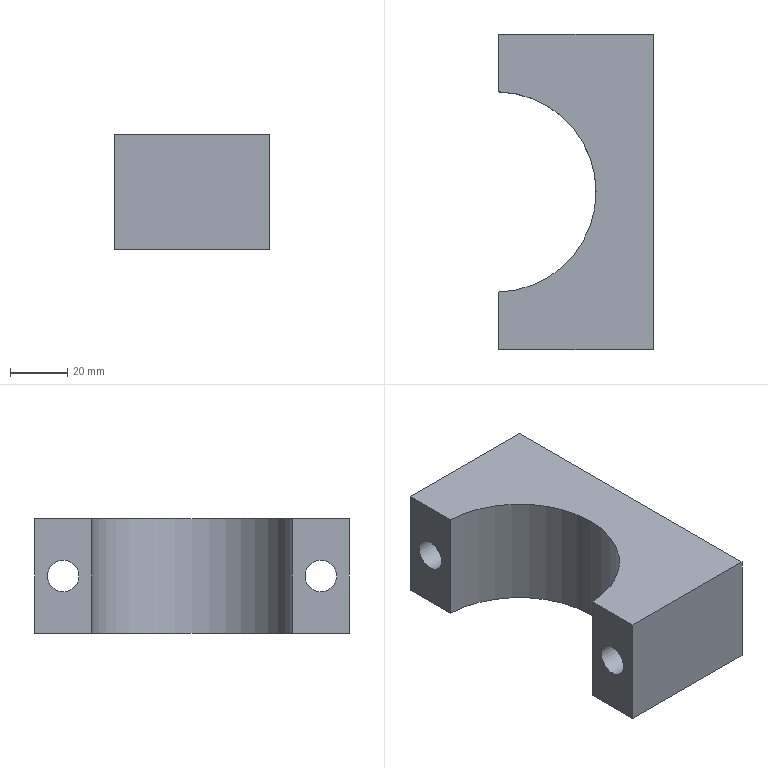Component | NX | CH3404_2-2 | 1 solid | 14 faces | box 54 x 110 x 40 mm | volume 151989 mm3 | plane 9 | cylinder 5 | commonest cylinder face diameters 11 x2 14 x2 70 x1
STEP:
#1=CARTESIAN_POINT('',(0.,0.,0.));
#2=DIRECTION('',(0.,0.,1.));
#3=DIRECTION('',(1.,0.,0.));
#4=AXIS2_PLACEMENT_3D('',#1,#2,#3);
#5=CARTESIAN_POINT('',(119.,-39.5,0.));
#6=VERTEX_POINT('',#5);
#7=CARTESIAN_POINT('',(119.,-50.5,0.));
#8=VERTEX_POINT('',#7);
#9=CARTESIAN_POINT('',(119.,-45.,0.));
#10=DIRECTION('',(1.,0.,0.));
#11=DIRECTION('',(-0.,1.,0.));
#12=AXIS2_PLACEMENT_3D('',#9,#10,#11);
#13=CIRCLE('',#12,5.5);
#14=CARTESIAN_POINT('',(119.,-34.986,20.));
#15=DIRECTION('',(1.,0.,0.));
#16=DIRECTION('',(-0.,1.,0.));
#17=AXIS2_PLACEMENT_3D('',#14,#15,#16);
#18=PLANE('',#17);
#19=CARTESIAN_POINT('',(-10.014,-20.));
#20=DIRECTION('',(1.,0.));
#21=AXIS2_PLACEMENT_2D('',#19,#20);
#22=CIRCLE('',#21,5.5);
#23=(GEOMETRIC_REPRESENTATION_CONTEXT(2)PARAMETRIC_REPRESENTATION_CONTEXT()REPRESENTATION_CONTEXT('',''));
#24=DEFINITIONAL_REPRESENTATION('',(#22),#23);
#25=PCURVE('',#18,#24);
#26=CARTESIAN_POINT('',(91.216,-45.,0.));
#27=DIRECTION('',(-1.,0.,0.));
#28=DIRECTION('',(-0.,-1.,0.));
#29=AXIS2_PLACEMENT_3D('',#26,#27,#28);
#30=CYLINDRICAL_SURFACE('',#29,5.5);
#31=CARTESIAN_POINT('',(3.142,-27.784));
#32=DIRECTION('',(-1.,0.));
#33=VECTOR('',#32,1.);
#34=LINE('',#31,#33);
#35=(GEOMETRIC_REPRESENTATION_CONTEXT(2)PARAMETRIC_REPRESENTATION_CONTEXT()REPRESENTATION_CONTEXT('',''));
#36=DEFINITIONAL_REPRESENTATION('',(#34),#35);
#37=PCURVE('',#30,#36);
#38=SURFACE_CURVE('',#13,(#25,#37),.PCURVE_S1.);
#39=EDGE_CURVE('',#6,#8,#38,.T.);
#40=ORIENTED_EDGE('',*,*,#39,.T.);
#41=CARTESIAN_POINT('',(119.,-45.,0.));
#42=DIRECTION('',(1.,0.,0.));
#43=DIRECTION('',(-0.,1.,0.));
#44=AXIS2_PLACEMENT_3D('',#41,#42,#43);
#45=CIRCLE('',#44,5.5);
#46=CARTESIAN_POINT('',(-10.014,-20.));
#47=DIRECTION('',(1.,0.));
#48=AXIS2_PLACEMENT_2D('',#46,#47);
#49=CIRCLE('',#48,5.5);
#50=(GEOMETRIC_REPRESENTATION_CONTEXT(2)PARAMETRIC_REPRESENTATION_CONTEXT()REPRESENTATION_CONTEXT('',''));
#51=DEFINITIONAL_REPRESENTATION('',(#49),#50);
#52=PCURVE('',#18,#51);
#53=CARTESIAN_POINT('',(9.425,-27.784));
#54=DIRECTION('',(-1.,0.));
#55=VECTOR('',#54,1.);
#56=LINE('',#53,#55);
#57=(GEOMETRIC_REPRESENTATION_CONTEXT(2)PARAMETRIC_REPRESENTATION_CONTEXT()REPRESENTATION_CONTEXT('',''));
#58=DEFINITIONAL_REPRESENTATION('',(#56),#57);
#59=PCURVE('',#30,#58);
#60=SURFACE_CURVE('',#45,(#52,#59),.PCURVE_S1.);
#61=EDGE_CURVE('',#8,#6,#60,.T.);
#62=ORIENTED_EDGE('',*,*,#61,.T.);
#63=EDGE_LOOP('',(#40,#62));
#64=FACE_BOUND('',#63,.T.);
#65=CARTESIAN_POINT('',(119.,-34.986,-20.));
#66=VERTEX_POINT('',#65);
#67=CARTESIAN_POINT('',(119.,-55.,-20.));
#68=VERTEX_POINT('',#67);
#69=CARTESIAN_POINT('',(119.,-34.986,-20.));
#70=DIRECTION('',(0.,-1.,0.));
#71=VECTOR('',#70,1.);
#72=LINE('',#69,#71);
#73=CARTESIAN_POINT('',(0.,-40.));
#74=DIRECTION('',(-1.,0.));
#75=VECTOR('',#74,1.);
#76=LINE('',#73,#75);
#77=(GEOMETRIC_REPRESENTATION_CONTEXT(2)PARAMETRIC_REPRESENTATION_CONTEXT()REPRESENTATION_CONTEXT('',''));
#78=DEFINITIONAL_REPRESENTATION('',(#76),#77);
#79=PCURVE('',#18,#78);
#80=CARTESIAN_POINT('',(118.,0.,-20.));
#81=DIRECTION('',(0.,0.,-1.));
#82=DIRECTION('',(-1.,0.,0.));
#83=AXIS2_PLACEMENT_3D('',#80,#81,#82);
#84=PLANE('',#83);
#85=CARTESIAN_POINT('',(-1.,-34.986));
#86=DIRECTION('',(-0.,-1.));
#87=VECTOR('',#86,1.);
#88=LINE('',#85,#87);
#89=(GEOMETRIC_REPRESENTATION_CONTEXT(2)PARAMETRIC_REPRESENTATION_CONTEXT()REPRESENTATION_CONTEXT('',''));
#90=DEFINITIONAL_REPRESENTATION('',(#88),#89);
#91=PCURVE('',#84,#90);
#92=SURFACE_CURVE('',#72,(#79,#91),.PCURVE_S1.);
#93=EDGE_CURVE('',#66,#68,#92,.T.);
#94=ORIENTED_EDGE('',*,*,#93,.T.);
#95=CARTESIAN_POINT('',(119.,-55.,20.));
#96=VERTEX_POINT('',#95);
#97=CARTESIAN_POINT('',(119.,-55.,20.));
#98=DIRECTION('',(0.,0.,-1.));
#99=VECTOR('',#98,1.);
#100=LINE('',#97,#99);
#101=CARTESIAN_POINT('',(-20.014,0.));
#102=DIRECTION('',(0.,-1.));
#103=VECTOR('',#102,1.);
#104=LINE('',#101,#103);
#105=(GEOMETRIC_REPRESENTATION_CONTEXT(2)PARAMETRIC_REPRESENTATION_CONTEXT()REPRESENTATION_CONTEXT('',''));
#106=DEFINITIONAL_REPRESENTATION('',(#104),#105);
#107=PCURVE('',#18,#106);
#108=CARTESIAN_POINT('',(119.,-55.,20.));
#109=DIRECTION('',(-0.,1.,0.));
#110=DIRECTION('',(-1.,-0.,0.));
#111=AXIS2_PLACEMENT_3D('',#108,#109,#110);
#112=PLANE('',#111);
#113=CARTESIAN_POINT('',(0.,0.));
#114=DIRECTION('',(0.,-1.));
#115=VECTOR('',#114,1.);
#116=LINE('',#113,#115);
#117=(GEOMETRIC_REPRESENTATION_CONTEXT(2)PARAMETRIC_REPRESENTATION_CONTEXT()REPRESENTATION_CONTEXT('',''));
#118=DEFINITIONAL_REPRESENTATION('',(#116),#117);
#119=PCURVE('',#112,#118);
#120=SURFACE_CURVE('',#100,(#107,#119),.PCURVE_S1.);
#121=EDGE_CURVE('',#96,#68,#120,.T.);
#122=ORIENTED_EDGE('',*,*,#121,.F.);
#123=CARTESIAN_POINT('',(119.,-34.986,20.));
#124=VERTEX_POINT('',#123);
#125=CARTESIAN_POINT('',(119.,-34.986,20.));
#126=DIRECTION('',(0.,-1.,0.));
#127=VECTOR('',#126,1.);
#128=LINE('',#125,#127);
#129=CARTESIAN_POINT('',(0.,0.));
#130=DIRECTION('',(-1.,0.));
#131=VECTOR('',#130,1.);
#132=LINE('',#129,#131);
#133=(GEOMETRIC_REPRESENTATION_CONTEXT(2)PARAMETRIC_REPRESENTATION_CONTEXT()REPRESENTATION_CONTEXT('',''));
#134=DEFINITIONAL_REPRESENTATION('',(#132),#133);
#135=PCURVE('',#18,#134);
#136=CARTESIAN_POINT('',(118.,0.,20.));
#137=DIRECTION('',(0.,0.,-1.));
#138=DIRECTION('',(-1.,0.,0.));
#139=AXIS2_PLACEMENT_3D('',#136,#137,#138);
#140=PLANE('',#139);
#141=CARTESIAN_POINT('',(-1.,-34.986));
#142=DIRECTION('',(-0.,-1.));
#143=VECTOR('',#142,1.);
#144=LINE('',#141,#143);
#145=(GEOMETRIC_REPRESENTATION_CONTEXT(2)PARAMETRIC_REPRESENTATION_CONTEXT()REPRESENTATION_CONTEXT('',''));
#146=DEFINITIONAL_REPRESENTATION('',(#144),#145);
#147=PCURVE('',#140,#146);
#148=SURFACE_CURVE('',#128,(#135,#147),.PCURVE_S1.);
#149=EDGE_CURVE('',#124,#96,#148,.T.);
#150=ORIENTED_EDGE('',*,*,#149,.F.);
#151=CARTESIAN_POINT('',(119.,-34.986,20.));
#152=DIRECTION('',(0.,0.,-1.));
#153=VECTOR('',#152,1.);
#154=LINE('',#151,#153);
#155=CARTESIAN_POINT('',(0.,0.));
#156=DIRECTION('',(0.,-1.));
#157=VECTOR('',#156,1.);
#158=LINE('',#155,#157);
#159=(GEOMETRIC_REPRESENTATION_CONTEXT(2)PARAMETRIC_REPRESENTATION_CONTEXT()REPRESENTATION_CONTEXT('',''));
#160=DEFINITIONAL_REPRESENTATION('',(#158),#159);
#161=PCURVE('',#18,#160);
#162=CARTESIAN_POINT('',(118.,0.,20.));
#163=DIRECTION('',(0.,0.,-1.));
#164=DIRECTION('',(-1.,0.,0.));
#165=AXIS2_PLACEMENT_3D('',#162,#163,#164);
#166=CYLINDRICAL_SURFACE('',#165,35.);
#167=CARTESIAN_POINT('',(4.684,0.));
#168=DIRECTION('',(0.,1.));
#169=VECTOR('',#168,1.);
#170=LINE('',#167,#169);
#171=(GEOMETRIC_REPRESENTATION_CONTEXT(2)PARAMETRIC_REPRESENTATION_CONTEXT()REPRESENTATION_CONTEXT('',''));
#172=DEFINITIONAL_REPRESENTATION('',(#170),#171);
#173=PCURVE('',#166,#172);
#174=SURFACE_CURVE('',#154,(#161,#173),.PCURVE_S1.);
#175=EDGE_CURVE('',#124,#66,#174,.T.);
#176=ORIENTED_EDGE('',*,*,#175,.T.);
#177=EDGE_LOOP('',(#94,#122,#150,#176));
#178=FACE_BOUND('',#177,.T.);
#179=ADVANCED_FACE('',(#64,#178),#18,.F.);
#180=CARTESIAN_POINT('',(173.,-55.,-20.));
#181=VERTEX_POINT('',#180);
#182=CARTESIAN_POINT('',(119.,-55.,-20.));
#183=DIRECTION('',(1.,0.,0.));
#184=VECTOR('',#183,1.);
#185=LINE('',#182,#184);
#186=CARTESIAN_POINT('',(0.,-40.));
#187=DIRECTION('',(-1.,0.));
#188=VECTOR('',#187,1.);
#189=LINE('',#186,#188);
#190=(GEOMETRIC_REPRESENTATION_CONTEXT(2)PARAMETRIC_REPRESENTATION_CONTEXT()REPRESENTATION_CONTEXT('',''));
#191=DEFINITIONAL_REPRESENTATION('',(#189),#190);
#192=PCURVE('',#112,#191);
#193=CARTESIAN_POINT('',(-1.,-55.));
#194=DIRECTION('',(-1.,0.));
#195=VECTOR('',#194,1.);
#196=LINE('',#193,#195);
#197=(GEOMETRIC_REPRESENTATION_CONTEXT(2)PARAMETRIC_REPRESENTATION_CONTEXT()REPRESENTATION_CONTEXT('',''));
#198=DEFINITIONAL_REPRESENTATION('',(#196),#197);
#199=PCURVE('',#84,#198);
#200=SURFACE_CURVE('',#185,(#192,#199),.PCURVE_S1.);
#201=EDGE_CURVE('',#68,#181,#200,.T.);
#202=ORIENTED_EDGE('',*,*,#201,.T.);
#203=CARTESIAN_POINT('',(173.,-55.,20.));
#204=VERTEX_POINT('',#203);
#205=CARTESIAN_POINT('',(173.,-55.,20.));
#206=DIRECTION('',(0.,0.,-1.));
#207=VECTOR('',#206,1.);
#208=LINE('',#205,#207);
#209=CARTESIAN_POINT('',(-54.,0.));
#210=DIRECTION('',(0.,-1.));
#211=VECTOR('',#210,1.);
#212=LINE('',#209,#211);
#213=(GEOMETRIC_REPRESENTATION_CONTEXT(2)PARAMETRIC_REPRESENTATION_CONTEXT()REPRESENTATION_CONTEXT('',''));
#214=DEFINITIONAL_REPRESENTATION('',(#212),#213);
#215=PCURVE('',#112,#214);
#216=CARTESIAN_POINT('',(173.,-55.,20.));
#217=DIRECTION('',(-1.,0.,0.));
#218=DIRECTION('',(-0.,-1.,0.));
#219=AXIS2_PLACEMENT_3D('',#216,#217,#218);
#220=PLANE('',#219);
#221=CARTESIAN_POINT('',(0.,0.));
#222=DIRECTION('',(0.,-1.));
#223=VECTOR('',#222,1.);
#224=LINE('',#221,#223);
#225=(GEOMETRIC_REPRESENTATION_CONTEXT(2)PARAMETRIC_REPRESENTATION_CONTEXT()REPRESENTATION_CONTEXT('',''));
#226=DEFINITIONAL_REPRESENTATION('',(#224),#225);
#227=PCURVE('',#220,#226);
#228=SURFACE_CURVE('',#208,(#215,#227),.PCURVE_S1.);
#229=EDGE_CURVE('',#204,#181,#228,.T.);
#230=ORIENTED_EDGE('',*,*,#229,.F.);
#231=CARTESIAN_POINT('',(119.,-55.,20.));
#232=DIRECTION('',(1.,0.,0.));
#233=VECTOR('',#232,1.);
#234=LINE('',#231,#233);
#235=CARTESIAN_POINT('',(0.,0.));
#236=DIRECTION('',(-1.,0.));
#237=VECTOR('',#236,1.);
#238=LINE('',#235,#237);
#239=(GEOMETRIC_REPRESENTATION_CONTEXT(2)PARAMETRIC_REPRESENTATION_CONTEXT()REPRESENTATION_CONTEXT('',''));
#240=DEFINITIONAL_REPRESENTATION('',(#238),#239);
#241=PCURVE('',#112,#240);
#242=CARTESIAN_POINT('',(-1.,-55.));
#243=DIRECTION('',(-1.,0.));
#244=VECTOR('',#243,1.);
#245=LINE('',#242,#244);
#246=(GEOMETRIC_REPRESENTATION_CONTEXT(2)PARAMETRIC_REPRESENTATION_CONTEXT()REPRESENTATION_CONTEXT('',''));
#247=DEFINITIONAL_REPRESENTATION('',(#245),#246);
#248=PCURVE('',#140,#247);
#249=SURFACE_CURVE('',#234,(#241,#248),.PCURVE_S1.);
#250=EDGE_CURVE('',#96,#204,#249,.T.);
#251=ORIENTED_EDGE('',*,*,#250,.F.);
#252=ORIENTED_EDGE('',*,*,#121,.T.);
#253=EDGE_LOOP('',(#202,#230,#251,#252));
#254=FACE_BOUND('',#253,.T.);
#255=ADVANCED_FACE('',(#254),#112,.F.);
#256=CARTESIAN_POINT('',(173.,38.,0.));
#257=VERTEX_POINT('',#256);
#258=CARTESIAN_POINT('',(173.,45.,0.));
#259=DIRECTION('',(-1.,0.,0.));
#260=DIRECTION('',(-0.,-1.,0.));
#261=AXIS2_PLACEMENT_3D('',#258,#259,#260);
#262=CIRCLE('',#261,7.);
#263=CARTESIAN_POINT('',(-100.,-20.));
#264=DIRECTION('',(1.,0.));
#265=AXIS2_PLACEMENT_2D('',#263,#264);
#266=CIRCLE('',#265,7.);
#267=(GEOMETRIC_REPRESENTATION_CONTEXT(2)PARAMETRIC_REPRESENTATION_CONTEXT()REPRESENTATION_CONTEXT('',''));
#268=DEFINITIONAL_REPRESENTATION('',(#266),#267);
#269=PCURVE('',#220,#268);
#270=CARTESIAN_POINT('',(173.,45.,0.));
#271=DIRECTION('',(-1.,0.,0.));
#272=DIRECTION('',(-0.,-1.,0.));
#273=AXIS2_PLACEMENT_3D('',#270,#271,#272);
#274=CYLINDRICAL_SURFACE('',#273,7.);
#275=CARTESIAN_POINT('',(0.,0.));
#276=DIRECTION('',(1.,0.));
#277=VECTOR('',#276,1.);
#278=LINE('',#275,#277);
#279=(GEOMETRIC_REPRESENTATION_CONTEXT(2)PARAMETRIC_REPRESENTATION_CONTEXT()REPRESENTATION_CONTEXT('',''));
#280=DEFINITIONAL_REPRESENTATION('',(#278),#279);
#281=PCURVE('',#274,#280);
#282=SURFACE_CURVE('',#262,(#269,#281),.PCURVE_S1.);
#283=EDGE_CURVE('',#257,#257,#282,.T.);
#284=ORIENTED_EDGE('',*,*,#283,.T.);
#285=EDGE_LOOP('',(#284));
#286=FACE_BOUND('',#285,.T.);
#287=CARTESIAN_POINT('',(173.,-52.,0.));
#288=VERTEX_POINT('',#287);
#289=CARTESIAN_POINT('',(173.,-45.,0.));
#290=DIRECTION('',(-1.,0.,0.));
#291=DIRECTION('',(-0.,-1.,0.));
#292=AXIS2_PLACEMENT_3D('',#289,#290,#291);
#293=CIRCLE('',#292,7.);
#294=CARTESIAN_POINT('',(-10.,-20.));
#295=DIRECTION('',(1.,0.));
#296=AXIS2_PLACEMENT_2D('',#294,#295);
#297=CIRCLE('',#296,7.);
#298=(GEOMETRIC_REPRESENTATION_CONTEXT(2)PARAMETRIC_REPRESENTATION_CONTEXT()REPRESENTATION_CONTEXT('',''));
#299=DEFINITIONAL_REPRESENTATION('',(#297),#298);
#300=PCURVE('',#220,#299);
#301=CARTESIAN_POINT('',(173.,-45.,0.));
#302=DIRECTION('',(-1.,0.,0.));
#303=DIRECTION('',(-0.,-1.,0.));
#304=AXIS2_PLACEMENT_3D('',#301,#302,#303);
#305=CYLINDRICAL_SURFACE('',#304,7.);
#306=CARTESIAN_POINT('',(0.,-0.));
#307=DIRECTION('',(1.,0.));
#308=VECTOR('',#307,1.);
#309=LINE('',#306,#308);
#310=(GEOMETRIC_REPRESENTATION_CONTEXT(2)PARAMETRIC_REPRESENTATION_CONTEXT()REPRESENTATION_CONTEXT('',''));
#311=DEFINITIONAL_REPRESENTATION('',(#309),#310);
#312=PCURVE('',#305,#311);
#313=SURFACE_CURVE('',#293,(#300,#312),.PCURVE_S1.);
#314=EDGE_CURVE('',#288,#288,#313,.T.);
#315=ORIENTED_EDGE('',*,*,#314,.T.);
#316=EDGE_LOOP('',(#315));
#317=FACE_BOUND('',#316,.T.);
#318=CARTESIAN_POINT('',(173.,55.,-20.));
#319=VERTEX_POINT('',#318);
#320=CARTESIAN_POINT('',(173.,-55.,-20.));
#321=DIRECTION('',(0.,1.,0.));
#322=VECTOR('',#321,1.);
#323=LINE('',#320,#322);
#324=CARTESIAN_POINT('',(0.,-40.));
#325=DIRECTION('',(-1.,0.));
#326=VECTOR('',#325,1.);
#327=LINE('',#324,#326);
#328=(GEOMETRIC_REPRESENTATION_CONTEXT(2)PARAMETRIC_REPRESENTATION_CONTEXT()REPRESENTATION_CONTEXT('',''));
#329=DEFINITIONAL_REPRESENTATION('',(#327),#328);
#330=PCURVE('',#220,#329);
#331=CARTESIAN_POINT('',(-55.,-55.));
#332=DIRECTION('',(-0.,1.));
#333=VECTOR('',#332,1.);
#334=LINE('',#331,#333);
#335=(GEOMETRIC_REPRESENTATION_CONTEXT(2)PARAMETRIC_REPRESENTATION_CONTEXT()REPRESENTATION_CONTEXT('',''));
#336=DEFINITIONAL_REPRESENTATION('',(#334),#335);
#337=PCURVE('',#84,#336);
#338=SURFACE_CURVE('',#323,(#330,#337),.PCURVE_S1.);
#339=EDGE_CURVE('',#181,#319,#338,.T.);
#340=ORIENTED_EDGE('',*,*,#339,.T.);
#341=CARTESIAN_POINT('',(173.,55.,20.));
#342=VERTEX_POINT('',#341);
#343=CARTESIAN_POINT('',(173.,55.,20.));
#344=DIRECTION('',(0.,0.,-1.));
#345=VECTOR('',#344,1.);
#346=LINE('',#343,#345);
#347=CARTESIAN_POINT('',(-110.,0.));
#348=DIRECTION('',(0.,-1.));
#349=VECTOR('',#348,1.);
#350=LINE('',#347,#349);
#351=(GEOMETRIC_REPRESENTATION_CONTEXT(2)PARAMETRIC_REPRESENTATION_CONTEXT()REPRESENTATION_CONTEXT('',''));
#352=DEFINITIONAL_REPRESENTATION('',(#350),#351);
#353=PCURVE('',#220,#352);
#354=CARTESIAN_POINT('',(173.,55.,20.));
#355=DIRECTION('',(-0.,-1.,0.));
#356=DIRECTION('',(1.,-0.,0.));
#357=AXIS2_PLACEMENT_3D('',#354,#355,#356);
#358=PLANE('',#357);
#359=CARTESIAN_POINT('',(0.,0.));
#360=DIRECTION('',(0.,-1.));
#361=VECTOR('',#360,1.);
#362=LINE('',#359,#361);
#363=(GEOMETRIC_REPRESENTATION_CONTEXT(2)PARAMETRIC_REPRESENTATION_CONTEXT()REPRESENTATION_CONTEXT('',''));
#364=DEFINITIONAL_REPRESENTATION('',(#362),#363);
#365=PCURVE('',#358,#364);
#366=SURFACE_CURVE('',#346,(#353,#365),.PCURVE_S1.);
#367=EDGE_CURVE('',#342,#319,#366,.T.);
#368=ORIENTED_EDGE('',*,*,#367,.F.);
#369=CARTESIAN_POINT('',(173.,-55.,20.));
#370=DIRECTION('',(0.,1.,0.));
#371=VECTOR('',#370,1.);
#372=LINE('',#369,#371);
#373=CARTESIAN_POINT('',(0.,0.));
#374=DIRECTION('',(-1.,0.));
#375=VECTOR('',#374,1.);
#376=LINE('',#373,#375);
#377=(GEOMETRIC_REPRESENTATION_CONTEXT(2)PARAMETRIC_REPRESENTATION_CONTEXT()REPRESENTATION_CONTEXT('',''));
#378=DEFINITIONAL_REPRESENTATION('',(#376),#377);
#379=PCURVE('',#220,#378);
#380=CARTESIAN_POINT('',(-55.,-55.));
#381=DIRECTION('',(-0.,1.));
#382=VECTOR('',#381,1.);
#383=LINE('',#380,#382);
#384=(GEOMETRIC_REPRESENTATION_CONTEXT(2)PARAMETRIC_REPRESENTATION_CONTEXT()REPRESENTATION_CONTEXT('',''));
#385=DEFINITIONAL_REPRESENTATION('',(#383),#384);
#386=PCURVE('',#140,#385);
#387=SURFACE_CURVE('',#372,(#379,#386),.PCURVE_S1.);
#388=EDGE_CURVE('',#204,#342,#387,.T.);
#389=ORIENTED_EDGE('',*,*,#388,.F.);
#390=ORIENTED_EDGE('',*,*,#229,.T.);
#391=EDGE_LOOP('',(#340,#368,#389,#390));
#392=FACE_BOUND('',#391,.T.);
#393=ADVANCED_FACE('',(#286,#317,#392),#220,.F.);
#394=CARTESIAN_POINT('',(119.,55.,-20.));
#395=VERTEX_POINT('',#394);
#396=CARTESIAN_POINT('',(173.,55.,-20.));
#397=DIRECTION('',(-1.,0.,0.));
#398=VECTOR('',#397,1.);
#399=LINE('',#396,#398);
#400=CARTESIAN_POINT('',(0.,-40.));
#401=DIRECTION('',(-1.,0.));
#402=VECTOR('',#401,1.);
#403=LINE('',#400,#402);
#404=(GEOMETRIC_REPRESENTATION_CONTEXT(2)PARAMETRIC_REPRESENTATION_CONTEXT()REPRESENTATION_CONTEXT('',''));
#405=DEFINITIONAL_REPRESENTATION('',(#403),#404);
#406=PCURVE('',#358,#405);
#407=CARTESIAN_POINT('',(-55.,55.));
#408=DIRECTION('',(1.,0.));
#409=VECTOR('',#408,1.);
#410=LINE('',#407,#409);
#411=(GEOMETRIC_REPRESENTATION_CONTEXT(2)PARAMETRIC_REPRESENTATION_CONTEXT()REPRESENTATION_CONTEXT('',''));
#412=DEFINITIONAL_REPRESENTATION('',(#410),#411);
#413=PCURVE('',#84,#412);
#414=SURFACE_CURVE('',#399,(#406,#413),.PCURVE_S1.);
#415=EDGE_CURVE('',#319,#395,#414,.T.);
#416=ORIENTED_EDGE('',*,*,#415,.T.);
#417=CARTESIAN_POINT('',(119.,55.,20.));
#418=VERTEX_POINT('',#417);
#419=CARTESIAN_POINT('',(119.,55.,20.));
#420=DIRECTION('',(0.,0.,-1.));
#421=VECTOR('',#420,1.);
#422=LINE('',#419,#421);
#423=CARTESIAN_POINT('',(-54.,0.));
#424=DIRECTION('',(0.,-1.));
#425=VECTOR('',#424,1.);
#426=LINE('',#423,#425);
#427=(GEOMETRIC_REPRESENTATION_CONTEXT(2)PARAMETRIC_REPRESENTATION_CONTEXT()REPRESENTATION_CONTEXT('',''));
#428=DEFINITIONAL_REPRESENTATION('',(#426),#427);
#429=PCURVE('',#358,#428);
#430=CARTESIAN_POINT('',(119.,55.,20.));
#431=DIRECTION('',(1.,-0.,0.));
#432=DIRECTION('',(0.,1.,0.));
#433=AXIS2_PLACEMENT_3D('',#430,#431,#432);
#434=PLANE('',#433);
#435=CARTESIAN_POINT('',(0.,0.));
#436=DIRECTION('',(0.,-1.));
#437=VECTOR('',#436,1.);
#438=LINE('',#435,#437);
#439=(GEOMETRIC_REPRESENTATION_CONTEXT(2)PARAMETRIC_REPRESENTATION_CONTEXT()REPRESENTATION_CONTEXT('',''));
#440=DEFINITIONAL_REPRESENTATION('',(#438),#439);
#441=PCURVE('',#434,#440);
#442=SURFACE_CURVE('',#422,(#429,#441),.PCURVE_S1.);
#443=EDGE_CURVE('',#418,#395,#442,.T.);
#444=ORIENTED_EDGE('',*,*,#443,.F.);
#445=CARTESIAN_POINT('',(173.,55.,20.));
#446=DIRECTION('',(-1.,0.,0.));
#447=VECTOR('',#446,1.);
#448=LINE('',#445,#447);
#449=CARTESIAN_POINT('',(0.,0.));
#450=DIRECTION('',(-1.,0.));
#451=VECTOR('',#450,1.);
#452=LINE('',#449,#451);
#453=(GEOMETRIC_REPRESENTATION_CONTEXT(2)PARAMETRIC_REPRESENTATION_CONTEXT()REPRESENTATION_CONTEXT('',''));
#454=DEFINITIONAL_REPRESENTATION('',(#452),#453);
#455=PCURVE('',#358,#454);
#456=CARTESIAN_POINT('',(-55.,55.));
#457=DIRECTION('',(1.,0.));
#458=VECTOR('',#457,1.);
#459=LINE('',#456,#458);
#460=(GEOMETRIC_REPRESENTATION_CONTEXT(2)PARAMETRIC_REPRESENTATION_CONTEXT()REPRESENTATION_CONTEXT('',''));
#461=DEFINITIONAL_REPRESENTATION('',(#459),#460);
#462=PCURVE('',#140,#461);
#463=SURFACE_CURVE('',#448,(#455,#462),.PCURVE_S1.);
#464=EDGE_CURVE('',#342,#418,#463,.T.);
#465=ORIENTED_EDGE('',*,*,#464,.F.);
#466=ORIENTED_EDGE('',*,*,#367,.T.);
#467=EDGE_LOOP('',(#416,#444,#465,#466));
#468=FACE_BOUND('',#467,.T.);
#469=ADVANCED_FACE('',(#468),#358,.F.);
#470=CARTESIAN_POINT('',(119.,50.5,0.));
#471=VERTEX_POINT('',#470);
#472=CARTESIAN_POINT('',(119.,39.5,0.));
#473=VERTEX_POINT('',#472);
#474=CARTESIAN_POINT('',(119.,45.,0.));
#475=DIRECTION('',(1.,-0.,0.));
#476=DIRECTION('',(0.,1.,0.));
#477=AXIS2_PLACEMENT_3D('',#474,#475,#476);
#478=CIRCLE('',#477,5.5);
#479=CARTESIAN_POINT('',(-10.,-20.));
#480=DIRECTION('',(1.,0.));
#481=AXIS2_PLACEMENT_2D('',#479,#480);
#482=CIRCLE('',#481,5.5);
#483=(GEOMETRIC_REPRESENTATION_CONTEXT(2)PARAMETRIC_REPRESENTATION_CONTEXT()REPRESENTATION_CONTEXT('',''));
#484=DEFINITIONAL_REPRESENTATION('',(#482),#483);
#485=PCURVE('',#434,#484);
#486=CARTESIAN_POINT('',(91.216,45.,0.));
#487=DIRECTION('',(-1.,0.,0.));
#488=DIRECTION('',(-0.,-1.,0.));
#489=AXIS2_PLACEMENT_3D('',#486,#487,#488);
#490=CYLINDRICAL_SURFACE('',#489,5.5);
#491=CARTESIAN_POINT('',(3.142,-27.784));
#492=DIRECTION('',(-1.,0.));
#493=VECTOR('',#492,1.);
#494=LINE('',#491,#493);
#495=(GEOMETRIC_REPRESENTATION_CONTEXT(2)PARAMETRIC_REPRESENTATION_CONTEXT()REPRESENTATION_CONTEXT('',''));
#496=DEFINITIONAL_REPRESENTATION('',(#494),#495);
#497=PCURVE('',#490,#496);
#498=SURFACE_CURVE('',#478,(#485,#497),.PCURVE_S1.);
#499=EDGE_CURVE('',#471,#473,#498,.T.);
#500=ORIENTED_EDGE('',*,*,#499,.T.);
#501=CARTESIAN_POINT('',(119.,45.,0.));
#502=DIRECTION('',(1.,-0.,0.));
#503=DIRECTION('',(0.,1.,0.));
#504=AXIS2_PLACEMENT_3D('',#501,#502,#503);
#505=CIRCLE('',#504,5.5);
#506=CARTESIAN_POINT('',(-10.,-20.));
#507=DIRECTION('',(1.,0.));
#508=AXIS2_PLACEMENT_2D('',#506,#507);
#509=CIRCLE('',#508,5.5);
#510=(GEOMETRIC_REPRESENTATION_CONTEXT(2)PARAMETRIC_REPRESENTATION_CONTEXT()REPRESENTATION_CONTEXT('',''));
#511=DEFINITIONAL_REPRESENTATION('',(#509),#510);
#512=PCURVE('',#434,#511);
#513=CARTESIAN_POINT('',(9.425,-27.784));
#514=DIRECTION('',(-1.,0.));
#515=VECTOR('',#514,1.);
#516=LINE('',#513,#515);
#517=(GEOMETRIC_REPRESENTATION_CONTEXT(2)PARAMETRIC_REPRESENTATION_CONTEXT()REPRESENTATION_CONTEXT('',''));
#518=DEFINITIONAL_REPRESENTATION('',(#516),#517);
#519=PCURVE('',#490,#518);
#520=SURFACE_CURVE('',#505,(#512,#519),.PCURVE_S1.);
#521=EDGE_CURVE('',#473,#471,#520,.T.);
#522=ORIENTED_EDGE('',*,*,#521,.T.);
#523=EDGE_LOOP('',(#500,#522));
#524=FACE_BOUND('',#523,.T.);
#525=CARTESIAN_POINT('',(119.,34.986,-20.));
#526=VERTEX_POINT('',#525);
#527=CARTESIAN_POINT('',(119.,55.,-20.));
#528=DIRECTION('',(-0.,-1.,0.));
#529=VECTOR('',#528,1.);
#530=LINE('',#527,#529);
#531=CARTESIAN_POINT('',(0.,-40.));
#532=DIRECTION('',(-1.,0.));
#533=VECTOR('',#532,1.);
#534=LINE('',#531,#533);
#535=(GEOMETRIC_REPRESENTATION_CONTEXT(2)PARAMETRIC_REPRESENTATION_CONTEXT()REPRESENTATION_CONTEXT('',''));
#536=DEFINITIONAL_REPRESENTATION('',(#534),#535);
#537=PCURVE('',#434,#536);
#538=CARTESIAN_POINT('',(-1.,55.));
#539=DIRECTION('',(0.,-1.));
#540=VECTOR('',#539,1.);
#541=LINE('',#538,#540);
#542=(GEOMETRIC_REPRESENTATION_CONTEXT(2)PARAMETRIC_REPRESENTATION_CONTEXT()REPRESENTATION_CONTEXT('',''));
#543=DEFINITIONAL_REPRESENTATION('',(#541),#542);
#544=PCURVE('',#84,#543);
#545=SURFACE_CURVE('',#530,(#537,#544),.PCURVE_S1.);
#546=EDGE_CURVE('',#395,#526,#545,.T.);
#547=ORIENTED_EDGE('',*,*,#546,.T.);
#548=CARTESIAN_POINT('',(119.,34.986,20.));
#549=VERTEX_POINT('',#548);
#550=CARTESIAN_POINT('',(119.,34.986,20.));
#551=DIRECTION('',(0.,0.,-1.));
#552=VECTOR('',#551,1.);
#553=LINE('',#550,#552);
#554=CARTESIAN_POINT('',(-20.014,0.));
#555=DIRECTION('',(0.,-1.));
#556=VECTOR('',#555,1.);
#557=LINE('',#554,#556);
#558=(GEOMETRIC_REPRESENTATION_CONTEXT(2)PARAMETRIC_REPRESENTATION_CONTEXT()REPRESENTATION_CONTEXT('',''));
#559=DEFINITIONAL_REPRESENTATION('',(#557),#558);
#560=PCURVE('',#434,#559);
#561=CARTESIAN_POINT('',(1.599,0.));
#562=DIRECTION('',(0.,1.));
#563=VECTOR('',#562,1.);
#564=LINE('',#561,#563);
#565=(GEOMETRIC_REPRESENTATION_CONTEXT(2)PARAMETRIC_REPRESENTATION_CONTEXT()REPRESENTATION_CONTEXT('',''));
#566=DEFINITIONAL_REPRESENTATION('',(#564),#565);
#567=PCURVE('',#166,#566);
#568=SURFACE_CURVE('',#553,(#560,#567),.PCURVE_S1.);
#569=EDGE_CURVE('',#549,#526,#568,.T.);
#570=ORIENTED_EDGE('',*,*,#569,.F.);
#571=CARTESIAN_POINT('',(119.,55.,20.));
#572=DIRECTION('',(-0.,-1.,0.));
#573=VECTOR('',#572,1.);
#574=LINE('',#571,#573);
#575=CARTESIAN_POINT('',(0.,0.));
#576=DIRECTION('',(-1.,0.));
#577=VECTOR('',#576,1.);
#578=LINE('',#575,#577);
#579=(GEOMETRIC_REPRESENTATION_CONTEXT(2)PARAMETRIC_REPRESENTATION_CONTEXT()REPRESENTATION_CONTEXT('',''));
#580=DEFINITIONAL_REPRESENTATION('',(#578),#579);
#581=PCURVE('',#434,#580);
#582=CARTESIAN_POINT('',(-1.,55.));
#583=DIRECTION('',(0.,-1.));
#584=VECTOR('',#583,1.);
#585=LINE('',#582,#584);
#586=(GEOMETRIC_REPRESENTATION_CONTEXT(2)PARAMETRIC_REPRESENTATION_CONTEXT()REPRESENTATION_CONTEXT('',''));
#587=DEFINITIONAL_REPRESENTATION('',(#585),#586);
#588=PCURVE('',#140,#587);
#589=SURFACE_CURVE('',#574,(#581,#588),.PCURVE_S1.);
#590=EDGE_CURVE('',#418,#549,#589,.T.);
#591=ORIENTED_EDGE('',*,*,#590,.F.);
#592=ORIENTED_EDGE('',*,*,#443,.T.);
#593=EDGE_LOOP('',(#547,#570,#591,#592));
#594=FACE_BOUND('',#593,.T.);
#595=ADVANCED_FACE('',(#524,#594),#434,.F.);
#596=ORIENTED_EDGE('',*,*,#569,.F.);
#597=CARTESIAN_POINT('',(118.,0.,20.));
#598=DIRECTION('',(0.,0.,-1.));
#599=DIRECTION('',(1.,0.,0.));
#600=AXIS2_PLACEMENT_3D('',#597,#598,#599);
#601=CIRCLE('',#600,35.);
#602=CARTESIAN_POINT('',(-3.142,0.));
#603=DIRECTION('',(1.,0.));
#604=VECTOR('',#603,1.);
#605=LINE('',#602,#604);
#606=(GEOMETRIC_REPRESENTATION_CONTEXT(2)PARAMETRIC_REPRESENTATION_CONTEXT()REPRESENTATION_CONTEXT('',''));
#607=DEFINITIONAL_REPRESENTATION('',(#605),#606);
#608=PCURVE('',#166,#607);
#609=CARTESIAN_POINT('',(0.,0.));
#610=DIRECTION('',(-1.,0.));
#611=AXIS2_PLACEMENT_2D('',#609,#610);
#612=CIRCLE('',#611,35.);
#613=(GEOMETRIC_REPRESENTATION_CONTEXT(2)PARAMETRIC_REPRESENTATION_CONTEXT()REPRESENTATION_CONTEXT('',''));
#614=DEFINITIONAL_REPRESENTATION('',(#612),#613);
#615=PCURVE('',#140,#614);
#616=SURFACE_CURVE('',#601,(#608,#615),.PCURVE_S1.);
#617=EDGE_CURVE('',#549,#124,#616,.T.);
#618=ORIENTED_EDGE('',*,*,#617,.T.);
#619=ORIENTED_EDGE('',*,*,#175,.T.);
#620=CARTESIAN_POINT('',(118.,0.,-20.));
#621=DIRECTION('',(0.,0.,-1.));
#622=DIRECTION('',(1.,0.,0.));
#623=AXIS2_PLACEMENT_3D('',#620,#621,#622);
#624=CIRCLE('',#623,35.);
#625=CARTESIAN_POINT('',(-3.142,40.));
#626=DIRECTION('',(1.,0.));
#627=VECTOR('',#626,1.);
#628=LINE('',#625,#627);
#629=(GEOMETRIC_REPRESENTATION_CONTEXT(2)PARAMETRIC_REPRESENTATION_CONTEXT()REPRESENTATION_CONTEXT('',''));
#630=DEFINITIONAL_REPRESENTATION('',(#628),#629);
#631=PCURVE('',#166,#630);
#632=CARTESIAN_POINT('',(0.,0.));
#633=DIRECTION('',(-1.,0.));
#634=AXIS2_PLACEMENT_2D('',#632,#633);
#635=CIRCLE('',#634,35.);
#636=(GEOMETRIC_REPRESENTATION_CONTEXT(2)PARAMETRIC_REPRESENTATION_CONTEXT()REPRESENTATION_CONTEXT('',''));
#637=DEFINITIONAL_REPRESENTATION('',(#635),#636);
#638=PCURVE('',#84,#637);
#639=SURFACE_CURVE('',#624,(#631,#638),.PCURVE_S1.);
#640=EDGE_CURVE('',#526,#66,#639,.T.);
#641=ORIENTED_EDGE('',*,*,#640,.F.);
#642=EDGE_LOOP('',(#596,#618,#619,#641));
#643=FACE_BOUND('',#642,.F.);
#644=ADVANCED_FACE('',(#643),#166,.F.);
#645=ORIENTED_EDGE('',*,*,#149,.T.);
#646=ORIENTED_EDGE('',*,*,#250,.T.);
#647=ORIENTED_EDGE('',*,*,#388,.T.);
#648=ORIENTED_EDGE('',*,*,#464,.T.);
#649=ORIENTED_EDGE('',*,*,#590,.T.);
#650=ORIENTED_EDGE('',*,*,#617,.T.);
#651=EDGE_LOOP('',(#645,#646,#647,#648,#649,#650));
#652=FACE_BOUND('',#651,.T.);
#653=ADVANCED_FACE('',(#652),#140,.F.);
#654=ORIENTED_EDGE('',*,*,#93,.F.);
#655=ORIENTED_EDGE('',*,*,#640,.F.);
#656=ORIENTED_EDGE('',*,*,#546,.F.);
#657=ORIENTED_EDGE('',*,*,#415,.F.);
#658=ORIENTED_EDGE('',*,*,#339,.F.);
#659=ORIENTED_EDGE('',*,*,#201,.F.);
#660=EDGE_LOOP('',(#654,#655,#656,#657,#658,#659));
#661=FACE_BOUND('',#660,.T.);
#662=ADVANCED_FACE('',(#661),#84,.T.);
#663=CARTESIAN_POINT('',(163.,-50.5,0.));
#664=VERTEX_POINT('',#663);
#665=CARTESIAN_POINT('',(163.,-45.,0.));
#666=DIRECTION('',(1.,-0.,0.));
#667=DIRECTION('',(-0.,-1.,0.));
#668=AXIS2_PLACEMENT_3D('',#665,#666,#667);
#669=CIRCLE('',#668,5.5);
#670=CARTESIAN_POINT('',(6.283,-71.784));
#671=DIRECTION('',(-1.,0.));
#672=VECTOR('',#671,1.);
#673=LINE('',#670,#672);
#674=(GEOMETRIC_REPRESENTATION_CONTEXT(2)PARAMETRIC_REPRESENTATION_CONTEXT()REPRESENTATION_CONTEXT('',''));
#675=DEFINITIONAL_REPRESENTATION('',(#673),#674);
#676=PCURVE('',#30,#675);
#677=CARTESIAN_POINT('',(163.,-45.,0.));
#678=DIRECTION('',(-1.,0.,0.));
#679=DIRECTION('',(-0.,-1.,0.));
#680=AXIS2_PLACEMENT_3D('',#677,#678,#679);
#681=PLANE('',#680);
#682=CARTESIAN_POINT('',(5.5,0.));
#683=CARTESIAN_POINT('',(5.5,-9.526));
#684=CARTESIAN_POINT('',(-2.75,-4.763));
#685=CARTESIAN_POINT('',(-11.,-0.));
#686=CARTESIAN_POINT('',(-2.75,4.763));
#687=CARTESIAN_POINT('',(5.5,9.526));
#688=CARTESIAN_POINT('',(5.5,0.));
#689=(BOUNDED_CURVE()B_SPLINE_CURVE(2,(#682,#683,#684,#685,#686,#687,#688),.UNSPECIFIED.,.T.,.F.)B_SPLINE_CURVE_WITH_KNOTS((1,2,2,2,2,1),(-2.094,0.,2.094,4.189,6.283,8.378),.UNSPECIFIED.)CURVE()GEOMETRIC_REPRESENTATION_ITEM()RATIONAL_B_SPLINE_CURVE((1.,0.5,1.,0.5,1.,0.5,1.))REPRESENTATION_ITEM(''));
#690=(GEOMETRIC_REPRESENTATION_CONTEXT(2)PARAMETRIC_REPRESENTATION_CONTEXT()REPRESENTATION_CONTEXT('',''));
#691=DEFINITIONAL_REPRESENTATION('',(#689),#690);
#692=PCURVE('',#681,#691);
#693=SURFACE_CURVE('',#669,(#676,#692),.PCURVE_S1.);
#694=EDGE_CURVE('',#664,#664,#693,.T.);
#695=ORIENTED_EDGE('',*,*,#694,.F.);
#696=CARTESIAN_POINT('',(163.,-50.5,0.));
#697=CARTESIAN_POINT('',(119.,-50.5,0.));
#698=B_SPLINE_CURVE_WITH_KNOTS('',1,(#696,#697),.UNSPECIFIED.,.F.,.F.,(2,2),(-71.784,-27.784),.PIECEWISE_BEZIER_KNOTS.);
#699=CARTESIAN_POINT('',(6.283,0.));
#700=DIRECTION('',(0.,1.));
#701=VECTOR('',#700,1.);
#702=LINE('',#699,#701);
#703=(GEOMETRIC_REPRESENTATION_CONTEXT(2)PARAMETRIC_REPRESENTATION_CONTEXT()REPRESENTATION_CONTEXT('',''));
#704=DEFINITIONAL_REPRESENTATION('',(#702),#703);
#705=PCURVE('',#30,#704);
#706=CARTESIAN_POINT('',(0.,0.));
#707=DIRECTION('',(0.,1.));
#708=VECTOR('',#707,1.);
#709=LINE('',#706,#708);
#710=(GEOMETRIC_REPRESENTATION_CONTEXT(2)PARAMETRIC_REPRESENTATION_CONTEXT()REPRESENTATION_CONTEXT('',''));
#711=DEFINITIONAL_REPRESENTATION('',(#709),#710);
#712=PCURVE('',#30,#711);
#713=SEAM_CURVE('',#698,(#705,#712),.PCURVE_S1.);
#714=EDGE_CURVE('',#664,#8,#713,.T.);
#715=ORIENTED_EDGE('',*,*,#714,.T.);
#716=ORIENTED_EDGE('',*,*,#61,.T.);
#717=ORIENTED_EDGE('',*,*,#39,.T.);
#718=ORIENTED_EDGE('',*,*,#714,.F.);
#719=EDGE_LOOP('',(#695,#715,#716,#717,#718));
#720=FACE_BOUND('',#719,.F.);
#721=ADVANCED_FACE('',(#720),#30,.F.);
#722=ORIENTED_EDGE('',*,*,#694,.F.);
#723=EDGE_LOOP('',(#722));
#724=FACE_BOUND('',#723,.T.);
#725=CARTESIAN_POINT('',(163.,-52.,0.));
#726=VERTEX_POINT('',#725);
#727=CARTESIAN_POINT('',(163.,-45.,0.));
#728=DIRECTION('',(1.,-0.,0.));
#729=DIRECTION('',(-0.,-1.,0.));
#730=AXIS2_PLACEMENT_3D('',#727,#728,#729);
#731=CIRCLE('',#730,7.);
#732=CARTESIAN_POINT('',(7.,0.));
#733=CARTESIAN_POINT('',(7.,-12.124));
#734=CARTESIAN_POINT('',(-3.5,-6.062));
#735=CARTESIAN_POINT('',(-14.,-0.));
#736=CARTESIAN_POINT('',(-3.5,6.062));
#737=CARTESIAN_POINT('',(7.,12.124));
#738=CARTESIAN_POINT('',(7.,0.));
#739=(BOUNDED_CURVE()B_SPLINE_CURVE(2,(#732,#733,#734,#735,#736,#737,#738),.UNSPECIFIED.,.T.,.F.)B_SPLINE_CURVE_WITH_KNOTS((1,2,2,2,2,1),(-2.094,0.,2.094,4.189,6.283,8.378),.UNSPECIFIED.)CURVE()GEOMETRIC_REPRESENTATION_ITEM()RATIONAL_B_SPLINE_CURVE((1.,0.5,1.,0.5,1.,0.5,1.))REPRESENTATION_ITEM(''));
#740=(GEOMETRIC_REPRESENTATION_CONTEXT(2)PARAMETRIC_REPRESENTATION_CONTEXT()REPRESENTATION_CONTEXT('',''));
#741=DEFINITIONAL_REPRESENTATION('',(#739),#740);
#742=PCURVE('',#681,#741);
#743=CARTESIAN_POINT('',(6.283,10.));
#744=DIRECTION('',(-1.,0.));
#745=VECTOR('',#744,1.);
#746=LINE('',#743,#745);
#747=(GEOMETRIC_REPRESENTATION_CONTEXT(2)PARAMETRIC_REPRESENTATION_CONTEXT()REPRESENTATION_CONTEXT('',''));
#748=DEFINITIONAL_REPRESENTATION('',(#746),#747);
#749=PCURVE('',#305,#748);
#750=SURFACE_CURVE('',#731,(#742,#749),.PCURVE_S1.);
#751=EDGE_CURVE('',#726,#726,#750,.T.);
#752=ORIENTED_EDGE('',*,*,#751,.T.);
#753=EDGE_LOOP('',(#752));
#754=FACE_BOUND('',#753,.T.);
#755=ADVANCED_FACE('',(#724,#754),#681,.F.);
#756=ORIENTED_EDGE('',*,*,#751,.T.);
#757=CARTESIAN_POINT('',(173.,-52.,0.));
#758=CARTESIAN_POINT('',(163.,-52.,0.));
#759=B_SPLINE_CURVE_WITH_KNOTS('',1,(#757,#758),.UNSPECIFIED.,.F.,.F.,(2,2),(-0.,10.),.PIECEWISE_BEZIER_KNOTS.);
#760=CARTESIAN_POINT('',(0.,0.));
#761=DIRECTION('',(0.,1.));
#762=VECTOR('',#761,1.);
#763=LINE('',#760,#762);
#764=(GEOMETRIC_REPRESENTATION_CONTEXT(2)PARAMETRIC_REPRESENTATION_CONTEXT()REPRESENTATION_CONTEXT('',''));
#765=DEFINITIONAL_REPRESENTATION('',(#763),#764);
#766=PCURVE('',#305,#765);
#767=CARTESIAN_POINT('',(6.283,0.));
#768=DIRECTION('',(0.,1.));
#769=VECTOR('',#768,1.);
#770=LINE('',#767,#769);
#771=(GEOMETRIC_REPRESENTATION_CONTEXT(2)PARAMETRIC_REPRESENTATION_CONTEXT()REPRESENTATION_CONTEXT('',''));
#772=DEFINITIONAL_REPRESENTATION('',(#770),#771);
#773=PCURVE('',#305,#772);
#774=SEAM_CURVE('',#759,(#766,#773),.PCURVE_S1.);
#775=EDGE_CURVE('',#288,#726,#774,.T.);
#776=ORIENTED_EDGE('',*,*,#775,.F.);
#777=ORIENTED_EDGE('',*,*,#314,.T.);
#778=ORIENTED_EDGE('',*,*,#775,.T.);
#779=EDGE_LOOP('',(#756,#776,#777,#778));
#780=FACE_BOUND('',#779,.F.);
#781=ADVANCED_FACE('',(#780),#305,.F.);
#782=CARTESIAN_POINT('',(163.,39.5,0.));
#783=VERTEX_POINT('',#782);
#784=CARTESIAN_POINT('',(163.,45.,0.));
#785=DIRECTION('',(1.,-0.,0.));
#786=DIRECTION('',(-0.,-1.,0.));
#787=AXIS2_PLACEMENT_3D('',#784,#785,#786);
#788=CIRCLE('',#787,5.5);
#789=CARTESIAN_POINT('',(6.283,-71.784));
#790=DIRECTION('',(-1.,0.));
#791=VECTOR('',#790,1.);
#792=LINE('',#789,#791);
#793=(GEOMETRIC_REPRESENTATION_CONTEXT(2)PARAMETRIC_REPRESENTATION_CONTEXT()REPRESENTATION_CONTEXT('',''));
#794=DEFINITIONAL_REPRESENTATION('',(#792),#793);
#795=PCURVE('',#490,#794);
#796=CARTESIAN_POINT('',(163.,45.,0.));
#797=DIRECTION('',(-1.,0.,0.));
#798=DIRECTION('',(-0.,-1.,0.));
#799=AXIS2_PLACEMENT_3D('',#796,#797,#798);
#800=PLANE('',#799);
#801=CARTESIAN_POINT('',(5.5,0.));
#802=CARTESIAN_POINT('',(5.5,-9.526));
#803=CARTESIAN_POINT('',(-2.75,-4.763));
#804=CARTESIAN_POINT('',(-11.,-0.));
#805=CARTESIAN_POINT('',(-2.75,4.763));
#806=CARTESIAN_POINT('',(5.5,9.526));
#807=CARTESIAN_POINT('',(5.5,0.));
#808=(BOUNDED_CURVE()B_SPLINE_CURVE(2,(#801,#802,#803,#804,#805,#806,#807),.UNSPECIFIED.,.T.,.F.)B_SPLINE_CURVE_WITH_KNOTS((1,2,2,2,2,1),(-2.094,0.,2.094,4.189,6.283,8.378),.UNSPECIFIED.)CURVE()GEOMETRIC_REPRESENTATION_ITEM()RATIONAL_B_SPLINE_CURVE((1.,0.5,1.,0.5,1.,0.5,1.))REPRESENTATION_ITEM(''));
#809=(GEOMETRIC_REPRESENTATION_CONTEXT(2)PARAMETRIC_REPRESENTATION_CONTEXT()REPRESENTATION_CONTEXT('',''));
#810=DEFINITIONAL_REPRESENTATION('',(#808),#809);
#811=PCURVE('',#800,#810);
#812=SURFACE_CURVE('',#788,(#795,#811),.PCURVE_S1.);
#813=EDGE_CURVE('',#783,#783,#812,.T.);
#814=ORIENTED_EDGE('',*,*,#813,.F.);
#815=CARTESIAN_POINT('',(163.,39.5,0.));
#816=CARTESIAN_POINT('',(119.,39.5,0.));
#817=B_SPLINE_CURVE_WITH_KNOTS('',1,(#815,#816),.UNSPECIFIED.,.F.,.F.,(2,2),(-71.784,-27.784),.PIECEWISE_BEZIER_KNOTS.);
#818=CARTESIAN_POINT('',(6.283,0.));
#819=DIRECTION('',(0.,1.));
#820=VECTOR('',#819,1.);
#821=LINE('',#818,#820);
#822=(GEOMETRIC_REPRESENTATION_CONTEXT(2)PARAMETRIC_REPRESENTATION_CONTEXT()REPRESENTATION_CONTEXT('',''));
#823=DEFINITIONAL_REPRESENTATION('',(#821),#822);
#824=PCURVE('',#490,#823);
#825=CARTESIAN_POINT('',(0.,0.));
#826=DIRECTION('',(0.,1.));
#827=VECTOR('',#826,1.);
#828=LINE('',#825,#827);
#829=(GEOMETRIC_REPRESENTATION_CONTEXT(2)PARAMETRIC_REPRESENTATION_CONTEXT()REPRESENTATION_CONTEXT('',''));
#830=DEFINITIONAL_REPRESENTATION('',(#828),#829);
#831=PCURVE('',#490,#830);
#832=SEAM_CURVE('',#817,(#824,#831),.PCURVE_S1.);
#833=EDGE_CURVE('',#783,#473,#832,.T.);
#834=ORIENTED_EDGE('',*,*,#833,.T.);
#835=ORIENTED_EDGE('',*,*,#521,.T.);
#836=ORIENTED_EDGE('',*,*,#499,.T.);
#837=ORIENTED_EDGE('',*,*,#833,.F.);
#838=EDGE_LOOP('',(#814,#834,#835,#836,#837));
#839=FACE_BOUND('',#838,.F.);
#840=ADVANCED_FACE('',(#839),#490,.F.);
#841=ORIENTED_EDGE('',*,*,#813,.F.);
#842=EDGE_LOOP('',(#841));
#843=FACE_BOUND('',#842,.T.);
#844=CARTESIAN_POINT('',(163.,38.,0.));
#845=VERTEX_POINT('',#844);
#846=CARTESIAN_POINT('',(163.,45.,0.));
#847=DIRECTION('',(1.,-0.,0.));
#848=DIRECTION('',(-0.,-1.,0.));
#849=AXIS2_PLACEMENT_3D('',#846,#847,#848);
#850=CIRCLE('',#849,7.);
#851=CARTESIAN_POINT('',(7.,0.));
#852=CARTESIAN_POINT('',(7.,-12.124));
#853=CARTESIAN_POINT('',(-3.5,-6.062));
#854=CARTESIAN_POINT('',(-14.,-0.));
#855=CARTESIAN_POINT('',(-3.5,6.062));
#856=CARTESIAN_POINT('',(7.,12.124));
#857=CARTESIAN_POINT('',(7.,0.));
#858=(BOUNDED_CURVE()B_SPLINE_CURVE(2,(#851,#852,#853,#854,#855,#856,#857),.UNSPECIFIED.,.T.,.F.)B_SPLINE_CURVE_WITH_KNOTS((1,2,2,2,2,1),(-2.094,0.,2.094,4.189,6.283,8.378),.UNSPECIFIED.)CURVE()GEOMETRIC_REPRESENTATION_ITEM()RATIONAL_B_SPLINE_CURVE((1.,0.5,1.,0.5,1.,0.5,1.))REPRESENTATION_ITEM(''));
#859=(GEOMETRIC_REPRESENTATION_CONTEXT(2)PARAMETRIC_REPRESENTATION_CONTEXT()REPRESENTATION_CONTEXT('',''));
#860=DEFINITIONAL_REPRESENTATION('',(#858),#859);
#861=PCURVE('',#800,#860);
#862=CARTESIAN_POINT('',(6.283,10.));
#863=DIRECTION('',(-1.,0.));
#864=VECTOR('',#863,1.);
#865=LINE('',#862,#864);
#866=(GEOMETRIC_REPRESENTATION_CONTEXT(2)PARAMETRIC_REPRESENTATION_CONTEXT()REPRESENTATION_CONTEXT('',''));
#867=DEFINITIONAL_REPRESENTATION('',(#865),#866);
#868=PCURVE('',#274,#867);
#869=SURFACE_CURVE('',#850,(#861,#868),.PCURVE_S1.);
#870=EDGE_CURVE('',#845,#845,#869,.T.);
#871=ORIENTED_EDGE('',*,*,#870,.T.);
#872=EDGE_LOOP('',(#871));
#873=FACE_BOUND('',#872,.T.);
#874=ADVANCED_FACE('',(#843,#873),#800,.F.);
#875=ORIENTED_EDGE('',*,*,#870,.T.);
#876=CARTESIAN_POINT('',(173.,38.,0.));
#877=CARTESIAN_POINT('',(163.,38.,0.));
#878=B_SPLINE_CURVE_WITH_KNOTS('',1,(#876,#877),.UNSPECIFIED.,.F.,.F.,(2,2),(0.,10.),.PIECEWISE_BEZIER_KNOTS.);
#879=CARTESIAN_POINT('',(0.,0.));
#880=DIRECTION('',(0.,1.));
#881=VECTOR('',#880,1.);
#882=LINE('',#879,#881);
#883=(GEOMETRIC_REPRESENTATION_CONTEXT(2)PARAMETRIC_REPRESENTATION_CONTEXT()REPRESENTATION_CONTEXT('',''));
#884=DEFINITIONAL_REPRESENTATION('',(#882),#883);
#885=PCURVE('',#274,#884);
#886=CARTESIAN_POINT('',(6.283,0.));
#887=DIRECTION('',(0.,1.));
#888=VECTOR('',#887,1.);
#889=LINE('',#886,#888);
#890=(GEOMETRIC_REPRESENTATION_CONTEXT(2)PARAMETRIC_REPRESENTATION_CONTEXT()REPRESENTATION_CONTEXT('',''));
#891=DEFINITIONAL_REPRESENTATION('',(#889),#890);
#892=PCURVE('',#274,#891);
#893=SEAM_CURVE('',#878,(#885,#892),.PCURVE_S1.);
#894=EDGE_CURVE('',#257,#845,#893,.T.);
#895=ORIENTED_EDGE('',*,*,#894,.F.);
#896=ORIENTED_EDGE('',*,*,#283,.T.);
#897=ORIENTED_EDGE('',*,*,#894,.T.);
#898=EDGE_LOOP('',(#875,#895,#896,#897));
#899=FACE_BOUND('',#898,.F.);
#900=ADVANCED_FACE('',(#899),#274,.F.);
#901=CLOSED_SHELL('',(#179,#255,#393,#469,#595,#644,#653,#662,#721,#755,#781,#840,#874,#900));
#902=MANIFOLD_SOLID_BREP('',#901);
#903=(LENGTH_UNIT()NAMED_UNIT(*)SI_UNIT(.MILLI.,.METRE.));
#904=UNCERTAINTY_MEASURE_WITH_UNIT(LENGTH_MEASURE(0.000002),#903,'','');
#905=(NAMED_UNIT(*)PLANE_ANGLE_UNIT()SI_UNIT($,.RADIAN.));
#906=(NAMED_UNIT(*)SI_UNIT($,.STERADIAN.)SOLID_ANGLE_UNIT());
#907=(GEOMETRIC_REPRESENTATION_CONTEXT(3)GLOBAL_UNCERTAINTY_ASSIGNED_CONTEXT((#904))GLOBAL_UNIT_ASSIGNED_CONTEXT((#903,#905,#906))REPRESENTATION_CONTEXT('',''));
#908=ADVANCED_BREP_SHAPE_REPRESENTATION('',(#4,#902),#907);